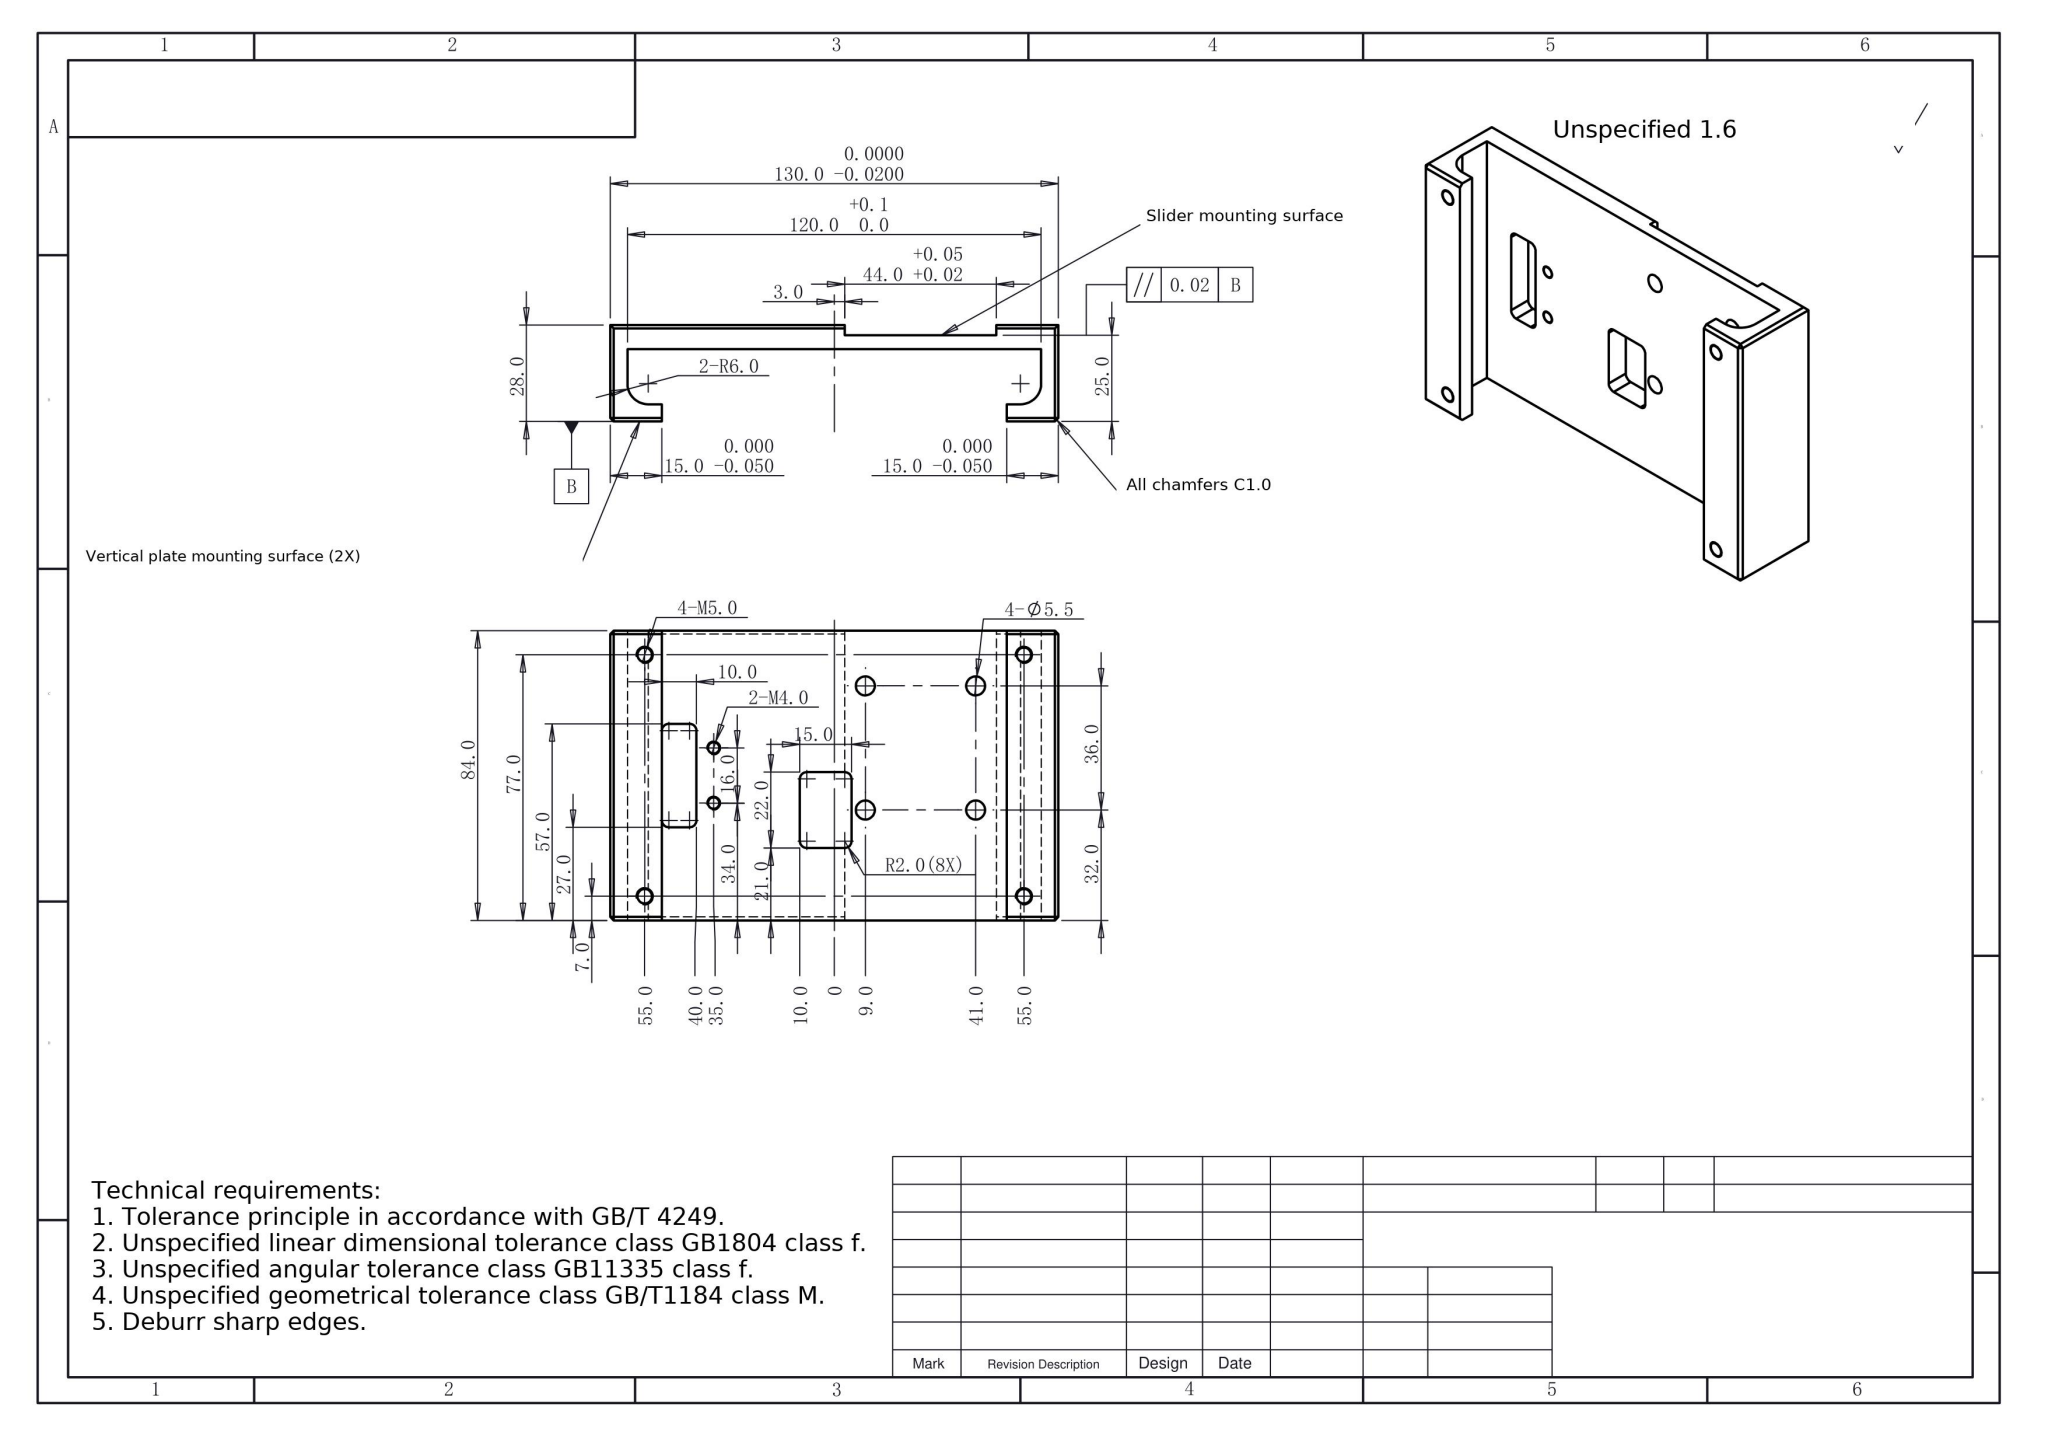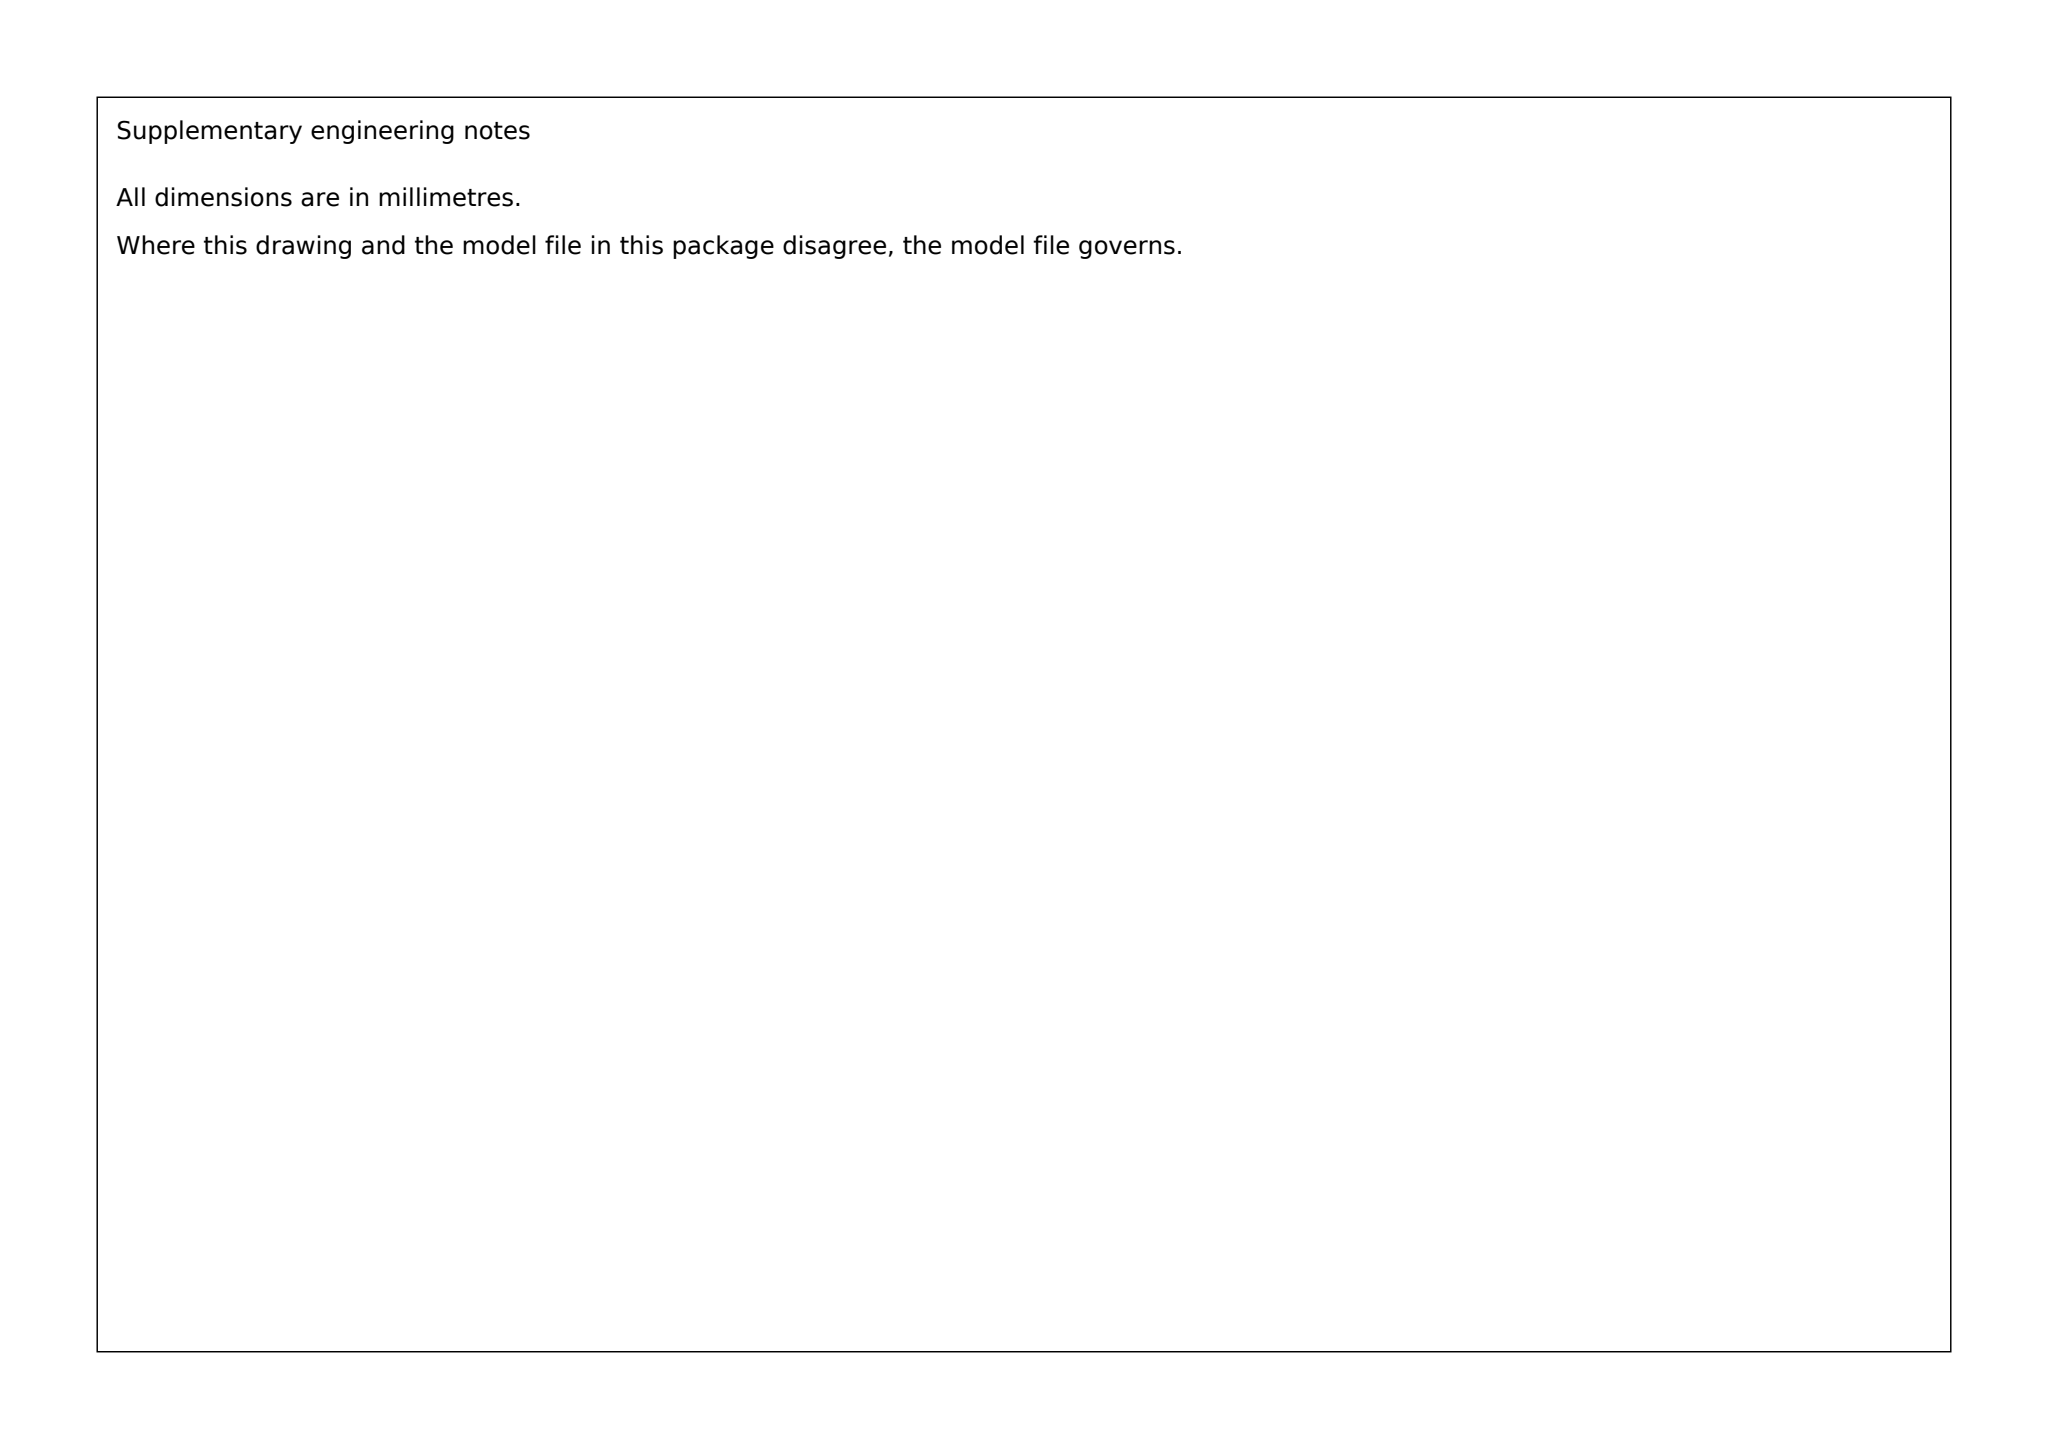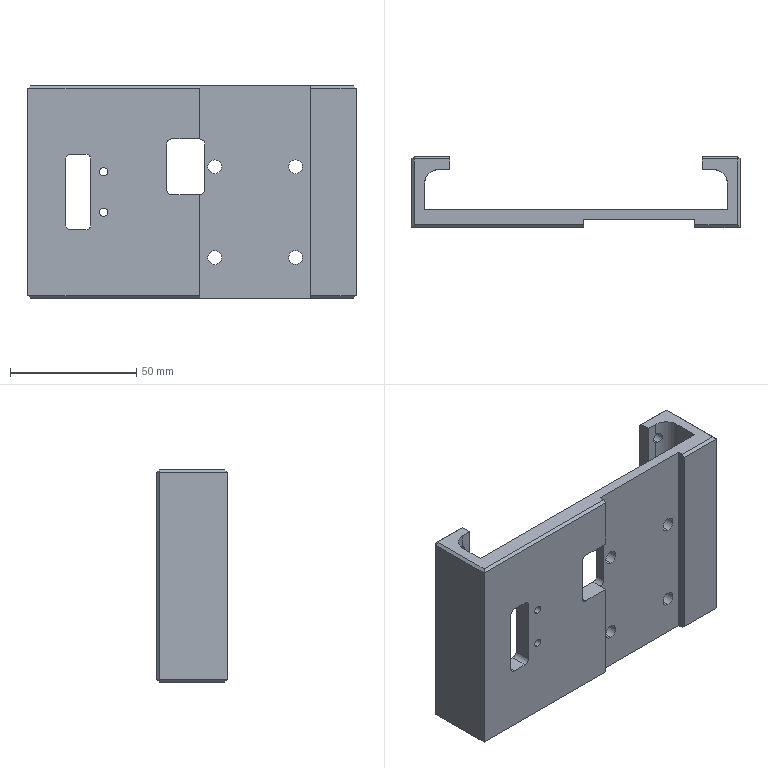Part | SolidWorks | mm | 1 solid | 75 faces | box 130 x 28 x 84 mm | volume 87416 mm3 | plane 45 | cylinder 30 | commonest cylinder face diameters 4.2 x8 5.5 x8 4 x8 3.3 x4 12 x2